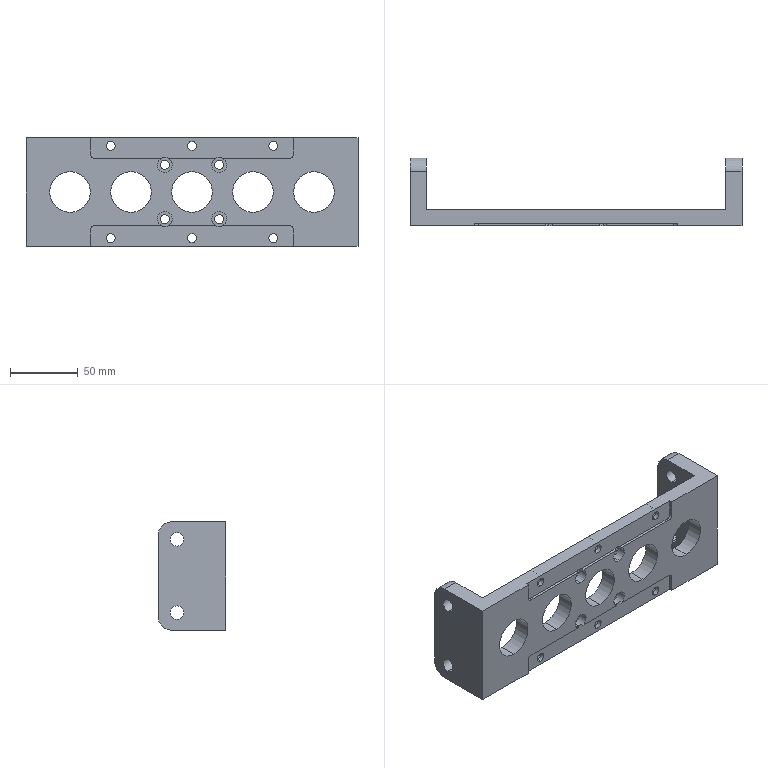Component | SolidWorks | ZTDJ-L-400-04-19-MaterialPortBagClamp-ConnectingRodSeat2-1 | 1 solid | 98 faces | box 245 x 50 x 80 mm | volume 244146 mm3 | cylinder 66 | plane 32 | commonest cylinder face diameters 11 x20 6.6 x20 30 x10 10 x8 20 x4 6 x4 | material 1023 Carbon Steel Sheet (SS)
build123d program:
from build123d import *

# Parameters (mm, degrees)
BOSS_EXTRUDE1_DEPTH                                  = 12
SKETCH2_W                                            = 80
SKETCH2_H                                            = 38
BOSS_EXTRUDE2_DEPTH                                  = 12
SKETCH3_R                                            = 5
CUT_EXTRUDE1_DEPTH                                   = 254.229
FILLET1_R                                            = 10
SKETCH6_W                                            = 150
SKETCH6_H                                            = 15
CUT_EXTRUDE3_DEPTH                                   = 2
FILLET2_R                                            = 3
SKETCH7_R                                            = 15
CUT_EXTRUDE4_DEPTH                                   = 139.225
LPATTERN1_COUNT                                      = 3
LPATTERN1_PITCH                                      = 45
LPATTERN2_COUNT                                      = 3
LPATTERN2_PITCH                                      = 45
HOLE_SIZE_ACCORDING_TO_THE_TYPE_OF_HEXAG_D           = 6.6
HOLE_SIZE_ACCORDING_TO_THE_TYPE_OF_HEXAG_CBORE_D     = 11
HOLE_SIZE_ACCORDING_TO_THE_TYPE_OF_HEXAG_CBORE_DEPTH = 6.8
HOLE_SIZE_ACCORDING_TO_THE_TYPE_OF_H_2_D             = 6.6
HOLE_SIZE_ACCORDING_TO_THE_TYPE_OF_H_2_CBORE_D       = 11
HOLE_SIZE_ACCORDING_TO_THE_TYPE_OF_H_2_CBORE_DEPTH   = 6.8


with BuildPart() as part:
    # Sketch1 → Boss-Extrude1 (new body)
    with BuildSketch(Plane(origin=(0, 0, 0), x_dir=(1, 0, 0), z_dir=(0, 1, 0))):
        Polygon((62.5, 40), (122.5, 40), (122.5, -40), (62.5, -40), (-122.5, -40), (-122.5, 40), align=None)
    extrude(amount=BOSS_EXTRUDE1_DEPTH)

    # Sketch2 → Boss-Extrude2 (add)
    with BuildSketch(Plane(origin=(122.5, 0, 0), x_dir=(0, 0, -1), z_dir=(1, 0, 0))):
        with Locations((0, 31)):
            Rectangle(SKETCH2_W, SKETCH2_H)
    boss_extrude2 = extrude(amount=-BOSS_EXTRUDE2_DEPTH)

    # Mirror1: Boss-Extrude2 across plane
    add(boss_extrude2.mirror(Plane(origin=(0, 0, 0), x_dir=(0, 0, 1), z_dir=(1, 0, 0))))

    # Sketch3 → Cut-Extrude1 (cut, through all)
    with BuildSketch(Plane(origin=(122.5, 0, 0), x_dir=(0, 0, -1), z_dir=(1, 0, 0))):
        with Locations((-27, 36)):
            Circle(SKETCH3_R)
        with Locations((27, 36)):
            Circle(SKETCH3_R)
    extrude(amount=-CUT_EXTRUDE1_DEPTH, mode=Mode.SUBTRACT)

    # Fillet1
    fillet1_edges = [part.edges().sort_by_distance(p)[0] for p in [
        (116.5, 50, -40),
        (116.5, 50, 40),
        (-116.5, 50, 40),
        (-116.5, 50, -40),
    ]]
    fillet(fillet1_edges, radius=FILLET1_R)

    # Sketch6 → Cut-Extrude3 (cut)
    with BuildSketch(Plane.XZ):
        with Locations((0, 32.5)):
            Rectangle(SKETCH6_W, SKETCH6_H)
        with Locations((0, -32.5)):
            Rectangle(SKETCH6_W, SKETCH6_H)
    extrude(amount=-CUT_EXTRUDE3_DEPTH, mode=Mode.SUBTRACT)

    # Fillet2
    fillet2_edges = [part.edges().sort_by_distance(p)[0] for p in [
        (-75, 1, 25),
        (-75, 1, -25),
        (75, 1, -25),
        (75, 1, 25),
    ]]
    fillet(fillet2_edges, radius=FILLET2_R)

    # Sketch7 → Cut-Extrude4 (cut, through all)
    with BuildSketch(Plane.XZ):
        with Locations(Location((0, 0, 0), (0, 0, 270))):
            Circle(SKETCH7_R)
    cut_extrude4 = extrude(amount=-CUT_EXTRUDE4_DEPTH, mode=Mode.SUBTRACT)

    # LPattern1: Cut-Extrude4 ×3
    with Locations(*[(i * LPATTERN1_PITCH, 0, 0) for i in range(1, LPATTERN1_COUNT)]):
        add(cut_extrude4, mode=Mode.SUBTRACT)

    # LPattern2: Cut-Extrude4 ×3
    with Locations(*[(-i * LPATTERN2_PITCH, 0, 0) for i in range(1, LPATTERN2_COUNT)]):
        add(cut_extrude4, mode=Mode.SUBTRACT)

    # Hole Size according to the type of Hexag (through all)
    with Locations(Plane(origin=(0, 12, 0), x_dir=(1, 0, 0), z_dir=(0, 1, 0))):
        with Locations((0, -34), (60, -34), (-60, -34)):
            hole_size_according_to_the_type_of_hexag = CounterBoreHole(HOLE_SIZE_ACCORDING_TO_THE_TYPE_OF_HEXAG_D / 2, HOLE_SIZE_ACCORDING_TO_THE_TYPE_OF_HEXAG_CBORE_D / 2, HOLE_SIZE_ACCORDING_TO_THE_TYPE_OF_HEXAG_CBORE_DEPTH)

    # Mirror2: Hole Size according to the type of Hexag across plane
    add(hole_size_according_to_the_type_of_hexag.mirror(Plane.XY), mode=Mode.SUBTRACT)

    # Hole Size according to the type of H 2 (through all)
    with Locations(Plane(origin=(0, 0, 0), x_dir=(-1, 0, 0), z_dir=(0, -1, 0))):
        with Locations((-20, 20), (-20, -20), (20, -20), (20, 20)):
            CounterBoreHole(HOLE_SIZE_ACCORDING_TO_THE_TYPE_OF_H_2_D / 2, HOLE_SIZE_ACCORDING_TO_THE_TYPE_OF_H_2_CBORE_D / 2, HOLE_SIZE_ACCORDING_TO_THE_TYPE_OF_H_2_CBORE_DEPTH)


solid = part.part

# Placed as in the assembly
solid = solid.moved(Location((-28.439, -46.186, 290), (0, 0, 0)))